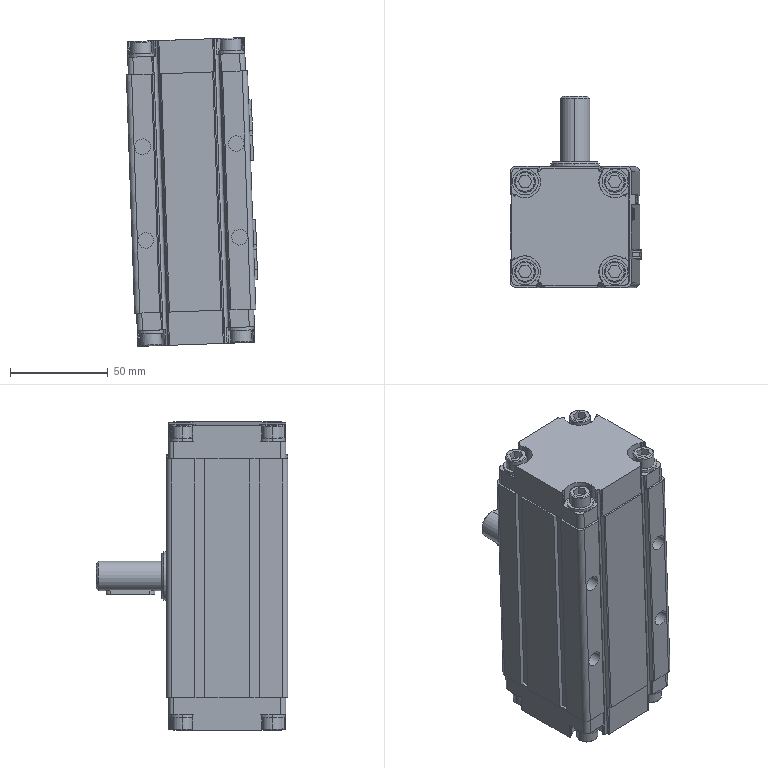Component | SolidWorks | RackAndPinionRotaryActuatorCDRA1BS50-180CZ-1 | 1 solid | 793 faces | box 67.2 x 98 x 158 mm | volume 575029 mm3 | plane 436 | cylinder 189 | spline 132 | torus 24 | sphere 8 | cone 4 | commonest cylinder face diameters 1.25 x56 2.5 x18 8 x16 10.667 x16 13.333 x16 16.281 x12 5.333 x12 8.5 x10